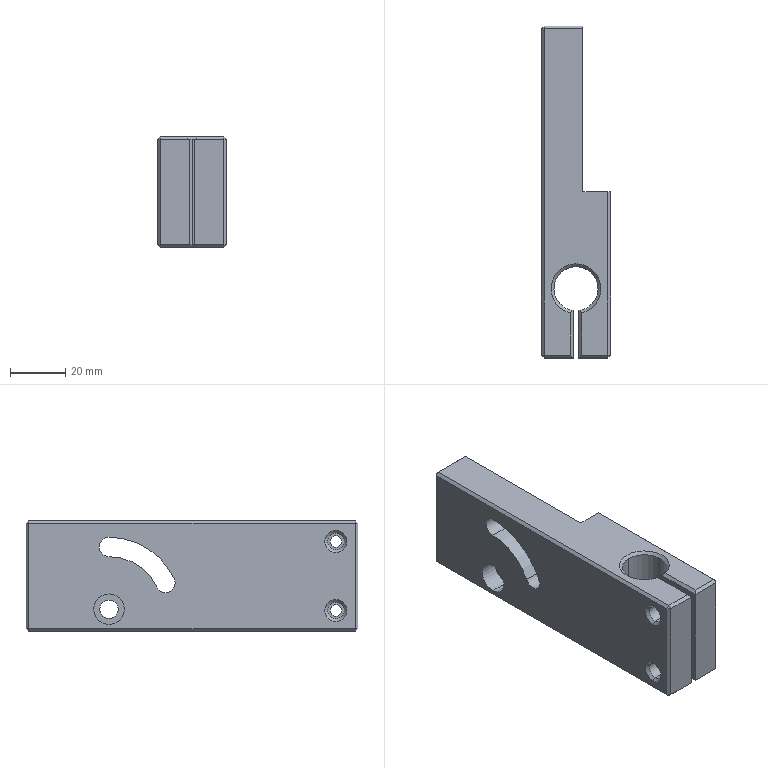Component | SolidWorks | CameraAssembly-1_GuideAxisFixingPlate-1 | 1 solid | 64 faces | box 25 x 120 x 40 mm | volume 81051 mm3 | plane 35 | cylinder 18 | cone 11 | commonest cylinder face diameters 4.2 x4 6 x4 11 x2 6.6 x2 16 x2 7 x2 52 x1 38 x1 | material 1060 Alloy
build123d program:
from build123d import *

# Parameters (mm, degrees)
SKETCH1_W                                          = 120
SKETCH1_H                                          = 25
BOSS_EXTRUDE1_DEPTH                                = 20
SKETCH2_R                                          = 8
CUT_EXTRUDE1_DEPTH                                 = 128.107
SKETCH3_W                                          = 19.536
SKETCH3_H                                          = 2
CUT_EXTRUDE2_DEPTH                                 = 128.107
SKETCH4_R                                          = 3
CUT_EXTRUDE3_DEPTH                                 = 11.5
M5_TAPPED_HOLE1_D                                  = 4.2
CHAMFER1_SIZE                                      = 1
SKETCH7_W                                          = 60
SKETCH7_H                                          = 21.078
CUT_EXTRUDE4_DEPTH                                 = 128.107
HOLE_SIZE_ACCORDING_TO_TYPE_OF_HEXAGON_D           = 6.6
HOLE_SIZE_ACCORDING_TO_TYPE_OF_HEXAGON_CBORE_D     = 11
HOLE_SIZE_ACCORDING_TO_TYPE_OF_HEXAGON_CBORE_DEPTH = 6.8
F_6_5_6_5_DIAMETER_HOLE1_D                         = 6.5
CUT_EXTRUDE5_DEPTH                                 = 125.197


with BuildPart() as part:
    # Sketch1 → Boss-Extrude1 (new, symmetric)
    with BuildSketch(Plane.XY):
        with Locations((60, 0)):
            Rectangle(SKETCH1_W, SKETCH1_H)
    extrude(amount=BOSS_EXTRUDE1_DEPTH, both=True)

    # Sketch2 → Cut-Extrude1 (cut, through all)
    with BuildSketch(Plane.XY.offset(20)):
        with Locations((25, 0)):
            Circle(SKETCH2_R)
    extrude(amount=-CUT_EXTRUDE1_DEPTH, mode=Mode.SUBTRACT)

    # Sketch3 → Cut-Extrude2 (cut, through all)
    with BuildSketch(Plane.XY.offset(20)):
        with Locations((9.768, 0)):
            Rectangle(SKETCH3_W, SKETCH3_H)
    extrude(amount=-CUT_EXTRUDE2_DEPTH, mode=Mode.SUBTRACT)

    # Sketch4 → Cut-Extrude3 (cut)
    with BuildSketch(Plane.XZ.offset(12.5)):
        with Locations(Location((8, 12.5, 0), (0, 0, 270))):
            Circle(SKETCH4_R)
        with Locations(Location((8, -12.5, 0), (0, 0, 270))):
            Circle(SKETCH4_R)
    extrude(amount=-CUT_EXTRUDE3_DEPTH, mode=Mode.SUBTRACT)

    # M5 Tapped Hole1 (through all)
    with Locations(Plane(origin=(0, 1, 0), x_dir=(-1, 0, 0), z_dir=(0, -1, 0))):
        with Locations((-8, 12.5), (-8, -12.5)):
            Hole(M5_TAPPED_HOLE1_D / 2)

    # Chamfer1
    chamfer1_edges = [part.edges().sort_by_distance(p)[0] for p in [
        (120, 0, 20),
        (60, 12.5, 20),
        (25.501, -7.984, -20),
        (25.501, 7.984, 20),
        (0, -6.75, -20),
        (0, -6.75, 20),
        (8.531, 1, -20),
        (8.531, -1, -20),
        (8.531, -1, 20),
        (8.531, 1, 20),
        (0, 6.75, 20),
        (8, -12.5, 15.5),
        (60, 12.5, -20),
        (8, -12.5, -9.5),
        (120, 0, -20),
        (60, -12.5, -20),
        (5.9, 12.5, 12.5),
        (0, 6.75, -20),
        (5.9, 12.5, -12.5),
        (60, -12.5, 20),
        (0, 12.5, 0),
        (120, 12.5, 0),
        (120, -12.5, 0),
        (0, -12.5, 0),
    ]]
    chamfer(chamfer1_edges, length=CHAMFER1_SIZE)

    # Sketch7 → Cut-Extrude4 (cut, through all)
    with BuildSketch(Plane.XY.offset(20)):
        with Locations((90, 13.039)):
            Rectangle(SKETCH7_W, SKETCH7_H)
    extrude(amount=-CUT_EXTRUDE4_DEPTH, mode=Mode.SUBTRACT)

    # Hole Size _according to_ type of Hexagon (through all)
    with Locations(Plane(origin=(0, -12.5, 0), x_dir=(-1, 0, 0), z_dir=(0, -1, 0))):
        with Locations((-90, -12)):
            CounterBoreHole(HOLE_SIZE_ACCORDING_TO_TYPE_OF_HEXAGON_D / 2, HOLE_SIZE_ACCORDING_TO_TYPE_OF_HEXAGON_CBORE_D / 2, HOLE_SIZE_ACCORDING_TO_TYPE_OF_HEXAGON_CBORE_DEPTH)

    # 6.5 _6.5_ Diameter Hole1 (through all)
    with Locations(Plane(origin=(0, -12.5, 0), x_dir=(-1, 0, 0), z_dir=(0, -1, 0))):
        with Locations((-77, 6.364)):
            Hole(F_6_5_6_5_DIAMETER_HOLE1_D / 2)

    # Sketch13 → Cut-Extrude5 (cut, through all)
    with BuildSketch(Plane.XZ.offset(12.5)):
        with BuildLine():
            ThreePointArc((72.78, 3.97), (79.791, -4.024), (90, -7))
            ThreePointArc((90, -7), (93.5, -10.5), (90, -14))
            ThreePointArc((90, -14), (76.03, -9.928), (66.436, 1.012))
            ThreePointArc((66.436, 1.012), (68.129, 5.663), (72.78, 3.97))
        make_face()
    extrude(amount=-CUT_EXTRUDE5_DEPTH, mode=Mode.SUBTRACT)


solid = part.part

# Placed as in the assembly
solid = solid.moved(Location((-119.666, 125.264, -287.5), (180, 0, -90)))